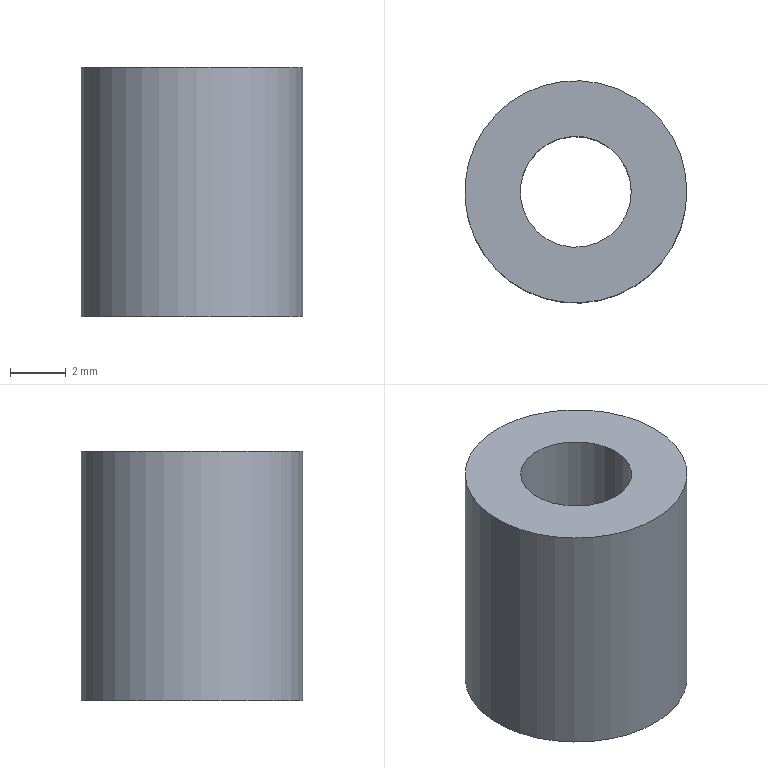Component | NX | FIXED_POST_2 | 1 solid | 4 faces | box 8 x 8 x 9 mm | volume 339 mm3 | cylinder 2 | plane 2 | commonest cylinder face diameters 8 x1 4 x1
STEP:
#1=CARTESIAN_POINT('',(0.,0.,0.));
#2=DIRECTION('',(0.,0.,1.));
#3=DIRECTION('',(1.,0.,0.));
#4=AXIS2_PLACEMENT_3D('',#1,#2,#3);
#5=CARTESIAN_POINT('',(236.5,-93.5,115.5));
#6=VERTEX_POINT('',#5);
#7=CARTESIAN_POINT('',(232.5,-93.5,115.5));
#8=DIRECTION('',(0.,0.,-1.));
#9=DIRECTION('',(1.,0.,0.));
#10=AXIS2_PLACEMENT_3D('',#7,#8,#9);
#11=CIRCLE('',#10,4.);
#12=CARTESIAN_POINT('',(232.5,-93.5,115.5));
#13=DIRECTION('',(0.,0.,-1.));
#14=DIRECTION('',(-1.,0.,0.));
#15=AXIS2_PLACEMENT_3D('',#12,#13,#14);
#16=CYLINDRICAL_SURFACE('',#15,4.);
#17=CARTESIAN_POINT('',(3.142,0.));
#18=DIRECTION('',(1.,0.));
#19=VECTOR('',#18,1.);
#20=LINE('',#17,#19);
#21=(GEOMETRIC_REPRESENTATION_CONTEXT(2)PARAMETRIC_REPRESENTATION_CONTEXT()REPRESENTATION_CONTEXT('',''));
#22=DEFINITIONAL_REPRESENTATION('',(#20),#21);
#23=PCURVE('',#16,#22);
#24=CARTESIAN_POINT('',(232.5,-93.5,115.5));
#25=DIRECTION('',(0.,0.,-1.));
#26=DIRECTION('',(-1.,0.,0.));
#27=AXIS2_PLACEMENT_3D('',#24,#25,#26);
#28=PLANE('',#27);
#29=CARTESIAN_POINT('',(0.,0.));
#30=DIRECTION('',(-1.,0.));
#31=AXIS2_PLACEMENT_2D('',#29,#30);
#32=CIRCLE('',#31,4.);
#33=(GEOMETRIC_REPRESENTATION_CONTEXT(2)PARAMETRIC_REPRESENTATION_CONTEXT()REPRESENTATION_CONTEXT('',''));
#34=DEFINITIONAL_REPRESENTATION('',(#32),#33);
#35=PCURVE('',#28,#34);
#36=SURFACE_CURVE('',#11,(#23,#35),.PCURVE_S1.);
#37=EDGE_CURVE('',#6,#6,#36,.T.);
#38=ORIENTED_EDGE('',*,*,#37,.T.);
#39=CARTESIAN_POINT('',(236.5,-93.5,106.5));
#40=VERTEX_POINT('',#39);
#41=CARTESIAN_POINT('',(236.5,-93.5,115.5));
#42=CARTESIAN_POINT('',(236.5,-93.5,106.5));
#43=B_SPLINE_CURVE_WITH_KNOTS('',1,(#41,#42),.UNSPECIFIED.,.F.,.F.,(2,2),(0.,9.),.PIECEWISE_BEZIER_KNOTS.);
#44=CARTESIAN_POINT('',(9.425,0.));
#45=DIRECTION('',(0.,1.));
#46=VECTOR('',#45,1.);
#47=LINE('',#44,#46);
#48=(GEOMETRIC_REPRESENTATION_CONTEXT(2)PARAMETRIC_REPRESENTATION_CONTEXT()REPRESENTATION_CONTEXT('',''));
#49=DEFINITIONAL_REPRESENTATION('',(#47),#48);
#50=PCURVE('',#16,#49);
#51=CARTESIAN_POINT('',(3.142,0.));
#52=DIRECTION('',(0.,1.));
#53=VECTOR('',#52,1.);
#54=LINE('',#51,#53);
#55=(GEOMETRIC_REPRESENTATION_CONTEXT(2)PARAMETRIC_REPRESENTATION_CONTEXT()REPRESENTATION_CONTEXT('',''));
#56=DEFINITIONAL_REPRESENTATION('',(#54),#55);
#57=PCURVE('',#16,#56);
#58=SEAM_CURVE('',#43,(#50,#57),.PCURVE_S1.);
#59=EDGE_CURVE('',#6,#40,#58,.T.);
#60=ORIENTED_EDGE('',*,*,#59,.T.);
#61=CARTESIAN_POINT('',(232.5,-93.5,106.5));
#62=DIRECTION('',(0.,0.,-1.));
#63=DIRECTION('',(1.,0.,0.));
#64=AXIS2_PLACEMENT_3D('',#61,#62,#63);
#65=CIRCLE('',#64,4.);
#66=CARTESIAN_POINT('',(3.142,9.));
#67=DIRECTION('',(1.,0.));
#68=VECTOR('',#67,1.);
#69=LINE('',#66,#68);
#70=(GEOMETRIC_REPRESENTATION_CONTEXT(2)PARAMETRIC_REPRESENTATION_CONTEXT()REPRESENTATION_CONTEXT('',''));
#71=DEFINITIONAL_REPRESENTATION('',(#69),#70);
#72=PCURVE('',#16,#71);
#73=CARTESIAN_POINT('',(232.5,-93.5,106.5));
#74=DIRECTION('',(0.,0.,-1.));
#75=DIRECTION('',(-1.,0.,0.));
#76=AXIS2_PLACEMENT_3D('',#73,#74,#75);
#77=PLANE('',#76);
#78=CARTESIAN_POINT('',(0.,0.));
#79=DIRECTION('',(-1.,0.));
#80=AXIS2_PLACEMENT_2D('',#78,#79);
#81=CIRCLE('',#80,4.);
#82=(GEOMETRIC_REPRESENTATION_CONTEXT(2)PARAMETRIC_REPRESENTATION_CONTEXT()REPRESENTATION_CONTEXT('',''));
#83=DEFINITIONAL_REPRESENTATION('',(#81),#82);
#84=PCURVE('',#77,#83);
#85=SURFACE_CURVE('',#65,(#72,#84),.PCURVE_S1.);
#86=EDGE_CURVE('',#40,#40,#85,.T.);
#87=ORIENTED_EDGE('',*,*,#86,.F.);
#88=ORIENTED_EDGE('',*,*,#59,.F.);
#89=EDGE_LOOP('',(#38,#60,#87,#88));
#90=FACE_BOUND('',#89,.T.);
#91=ADVANCED_FACE('',(#90),#16,.T.);
#92=CARTESIAN_POINT('',(234.5,-93.5,115.5));
#93=VERTEX_POINT('',#92);
#94=CARTESIAN_POINT('',(232.5,-93.5,115.5));
#95=DIRECTION('',(0.,0.,-1.));
#96=DIRECTION('',(1.,0.,0.));
#97=AXIS2_PLACEMENT_3D('',#94,#95,#96);
#98=CIRCLE('',#97,2.);
#99=CARTESIAN_POINT('',(232.5,-93.5,115.5));
#100=DIRECTION('',(0.,0.,-1.));
#101=DIRECTION('',(-1.,0.,0.));
#102=AXIS2_PLACEMENT_3D('',#99,#100,#101);
#103=CYLINDRICAL_SURFACE('',#102,2.);
#104=CARTESIAN_POINT('',(3.142,0.));
#105=DIRECTION('',(1.,0.));
#106=VECTOR('',#105,1.);
#107=LINE('',#104,#106);
#108=(GEOMETRIC_REPRESENTATION_CONTEXT(2)PARAMETRIC_REPRESENTATION_CONTEXT()REPRESENTATION_CONTEXT('',''));
#109=DEFINITIONAL_REPRESENTATION('',(#107),#108);
#110=PCURVE('',#103,#109);
#111=CARTESIAN_POINT('',(0.,0.));
#112=DIRECTION('',(-1.,0.));
#113=AXIS2_PLACEMENT_2D('',#111,#112);
#114=CIRCLE('',#113,2.);
#115=(GEOMETRIC_REPRESENTATION_CONTEXT(2)PARAMETRIC_REPRESENTATION_CONTEXT()REPRESENTATION_CONTEXT('',''));
#116=DEFINITIONAL_REPRESENTATION('',(#114),#115);
#117=PCURVE('',#28,#116);
#118=SURFACE_CURVE('',#98,(#110,#117),.PCURVE_S1.);
#119=EDGE_CURVE('',#93,#93,#118,.T.);
#120=ORIENTED_EDGE('',*,*,#119,.T.);
#121=CARTESIAN_POINT('',(234.5,-93.5,106.5));
#122=VERTEX_POINT('',#121);
#123=CARTESIAN_POINT('',(234.5,-93.5,115.5));
#124=CARTESIAN_POINT('',(234.5,-93.5,106.5));
#125=B_SPLINE_CURVE_WITH_KNOTS('',1,(#123,#124),.UNSPECIFIED.,.F.,.F.,(2,2),(0.,9.),.PIECEWISE_BEZIER_KNOTS.);
#126=CARTESIAN_POINT('',(9.425,0.));
#127=DIRECTION('',(0.,1.));
#128=VECTOR('',#127,1.);
#129=LINE('',#126,#128);
#130=(GEOMETRIC_REPRESENTATION_CONTEXT(2)PARAMETRIC_REPRESENTATION_CONTEXT()REPRESENTATION_CONTEXT('',''));
#131=DEFINITIONAL_REPRESENTATION('',(#129),#130);
#132=PCURVE('',#103,#131);
#133=CARTESIAN_POINT('',(3.142,0.));
#134=DIRECTION('',(0.,1.));
#135=VECTOR('',#134,1.);
#136=LINE('',#133,#135);
#137=(GEOMETRIC_REPRESENTATION_CONTEXT(2)PARAMETRIC_REPRESENTATION_CONTEXT()REPRESENTATION_CONTEXT('',''));
#138=DEFINITIONAL_REPRESENTATION('',(#136),#137);
#139=PCURVE('',#103,#138);
#140=SEAM_CURVE('',#125,(#132,#139),.PCURVE_S1.);
#141=EDGE_CURVE('',#93,#122,#140,.T.);
#142=ORIENTED_EDGE('',*,*,#141,.T.);
#143=CARTESIAN_POINT('',(232.5,-93.5,106.5));
#144=DIRECTION('',(0.,0.,-1.));
#145=DIRECTION('',(1.,0.,0.));
#146=AXIS2_PLACEMENT_3D('',#143,#144,#145);
#147=CIRCLE('',#146,2.);
#148=CARTESIAN_POINT('',(3.142,9.));
#149=DIRECTION('',(1.,0.));
#150=VECTOR('',#149,1.);
#151=LINE('',#148,#150);
#152=(GEOMETRIC_REPRESENTATION_CONTEXT(2)PARAMETRIC_REPRESENTATION_CONTEXT()REPRESENTATION_CONTEXT('',''));
#153=DEFINITIONAL_REPRESENTATION('',(#151),#152);
#154=PCURVE('',#103,#153);
#155=CARTESIAN_POINT('',(0.,0.));
#156=DIRECTION('',(-1.,0.));
#157=AXIS2_PLACEMENT_2D('',#155,#156);
#158=CIRCLE('',#157,2.);
#159=(GEOMETRIC_REPRESENTATION_CONTEXT(2)PARAMETRIC_REPRESENTATION_CONTEXT()REPRESENTATION_CONTEXT('',''));
#160=DEFINITIONAL_REPRESENTATION('',(#158),#159);
#161=PCURVE('',#77,#160);
#162=SURFACE_CURVE('',#147,(#154,#161),.PCURVE_S1.);
#163=EDGE_CURVE('',#122,#122,#162,.T.);
#164=ORIENTED_EDGE('',*,*,#163,.F.);
#165=ORIENTED_EDGE('',*,*,#141,.F.);
#166=EDGE_LOOP('',(#120,#142,#164,#165));
#167=FACE_BOUND('',#166,.F.);
#168=ADVANCED_FACE('',(#167),#103,.F.);
#169=ORIENTED_EDGE('',*,*,#37,.F.);
#170=EDGE_LOOP('',(#169));
#171=FACE_BOUND('',#170,.T.);
#172=ORIENTED_EDGE('',*,*,#119,.T.);
#173=EDGE_LOOP('',(#172));
#174=FACE_BOUND('',#173,.T.);
#175=ADVANCED_FACE('',(#171,#174),#28,.F.);
#176=ORIENTED_EDGE('',*,*,#86,.T.);
#177=EDGE_LOOP('',(#176));
#178=FACE_BOUND('',#177,.T.);
#179=ORIENTED_EDGE('',*,*,#163,.F.);
#180=EDGE_LOOP('',(#179));
#181=FACE_BOUND('',#180,.T.);
#182=ADVANCED_FACE('',(#178,#181),#77,.T.);
#183=CLOSED_SHELL('',(#91,#168,#175,#182));
#184=MANIFOLD_SOLID_BREP('',#183);
#185=(LENGTH_UNIT()NAMED_UNIT(*)SI_UNIT(.MILLI.,.METRE.));
#186=UNCERTAINTY_MEASURE_WITH_UNIT(LENGTH_MEASURE(0.00001),#185,'','');
#187=(NAMED_UNIT(*)PLANE_ANGLE_UNIT()SI_UNIT($,.RADIAN.));
#188=(NAMED_UNIT(*)SI_UNIT($,.STERADIAN.)SOLID_ANGLE_UNIT());
#189=(GEOMETRIC_REPRESENTATION_CONTEXT(3)GLOBAL_UNCERTAINTY_ASSIGNED_CONTEXT((#186))GLOBAL_UNIT_ASSIGNED_CONTEXT((#185,#187,#188))REPRESENTATION_CONTEXT('',''));
#190=ADVANCED_BREP_SHAPE_REPRESENTATION('',(#4,#184),#189);